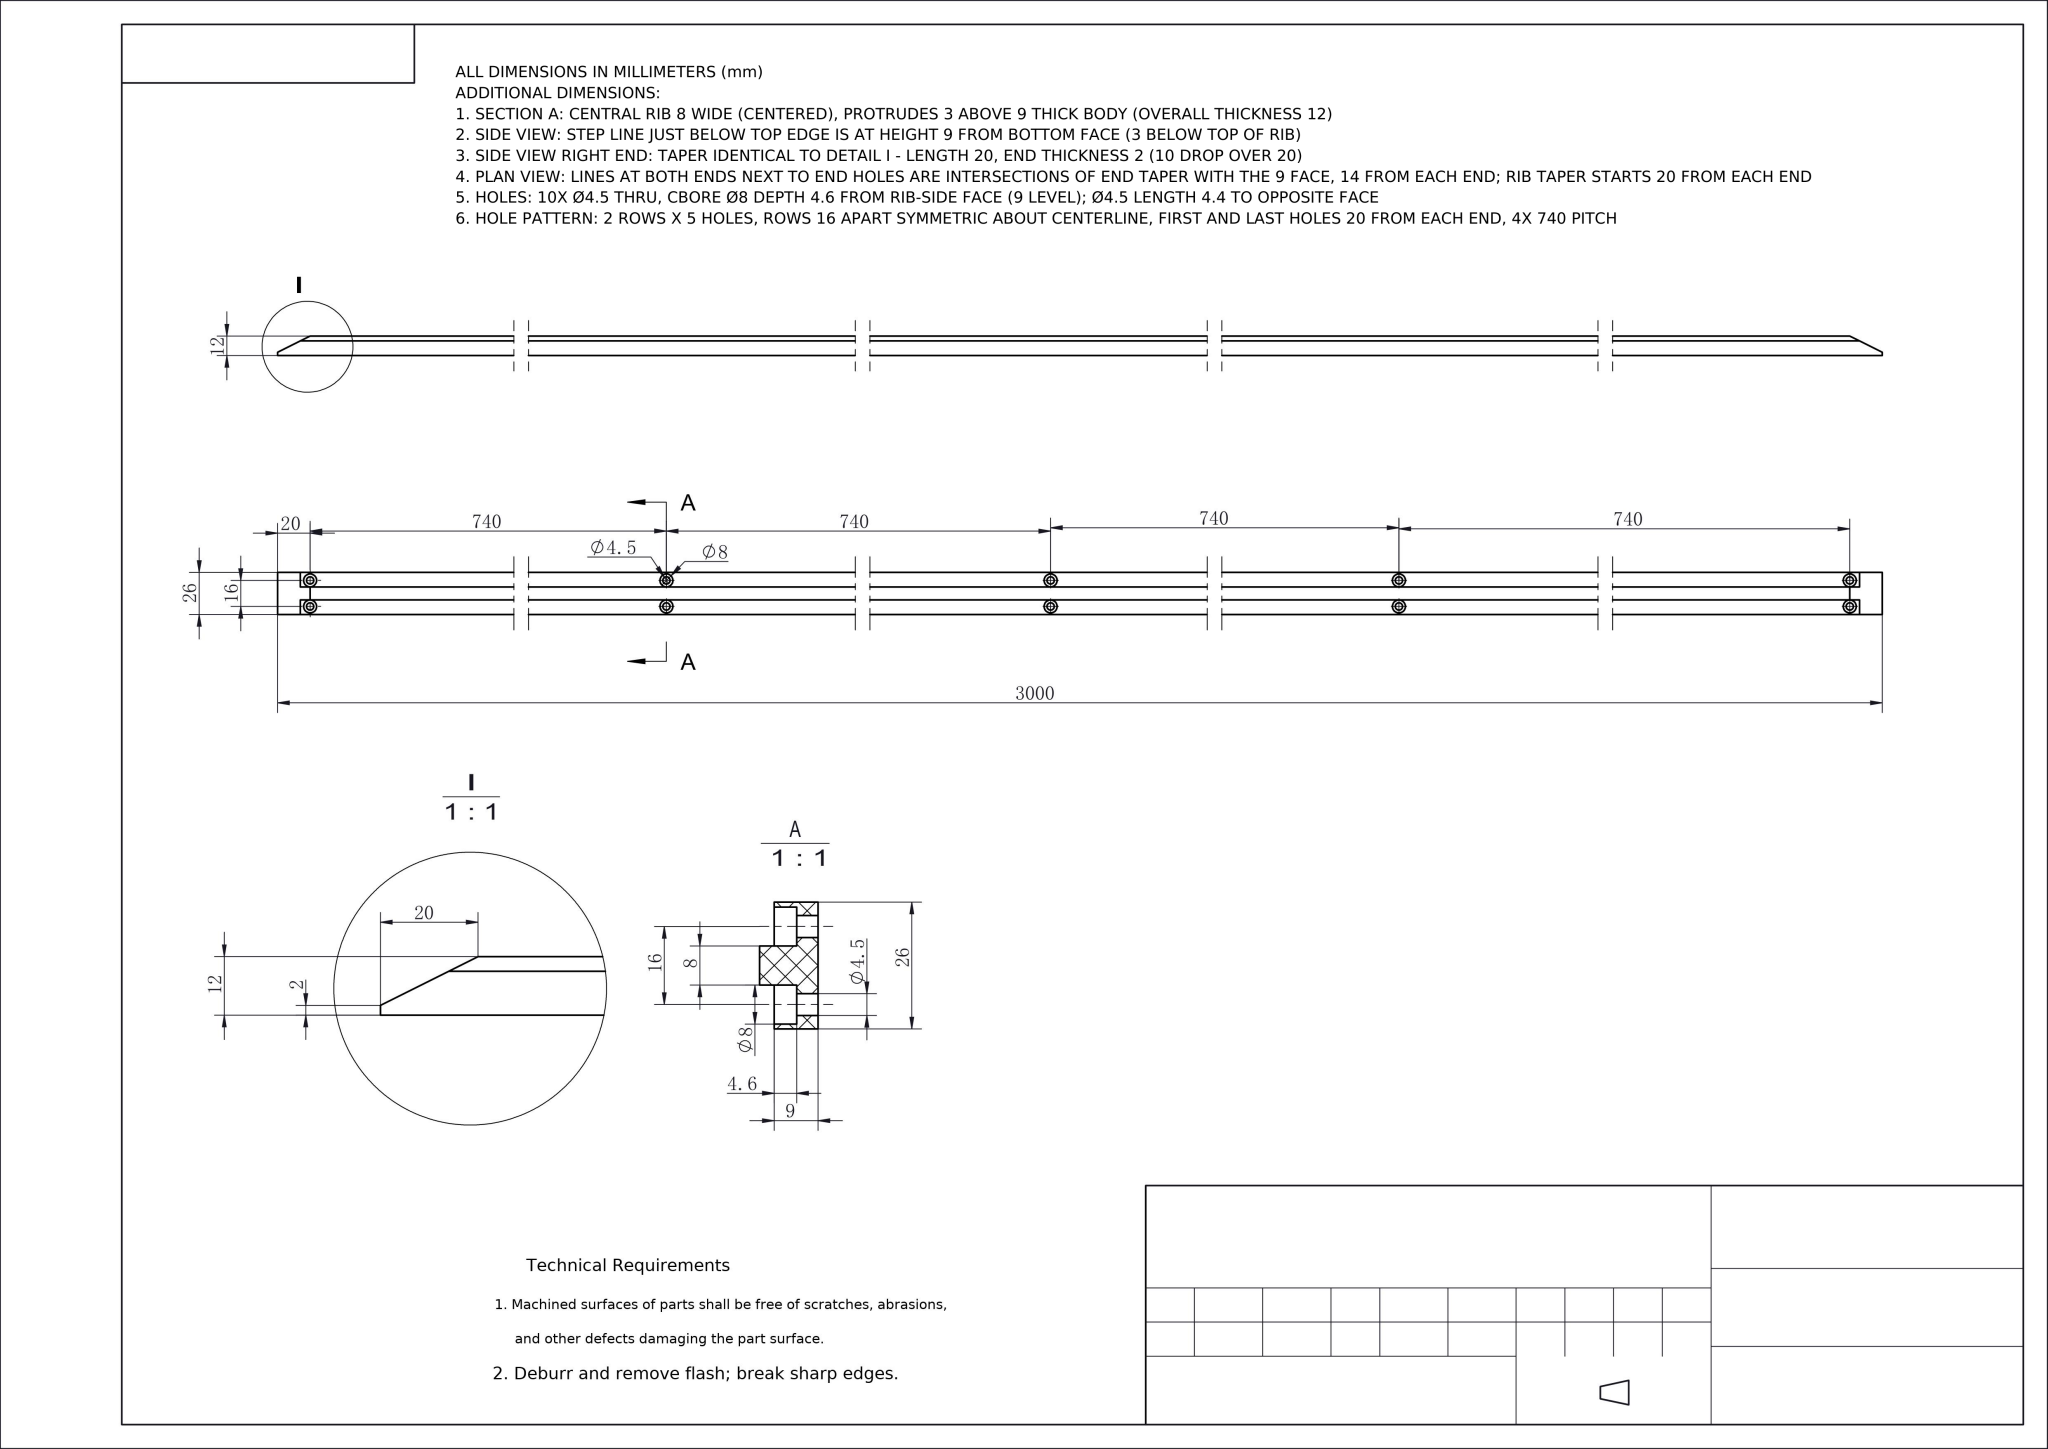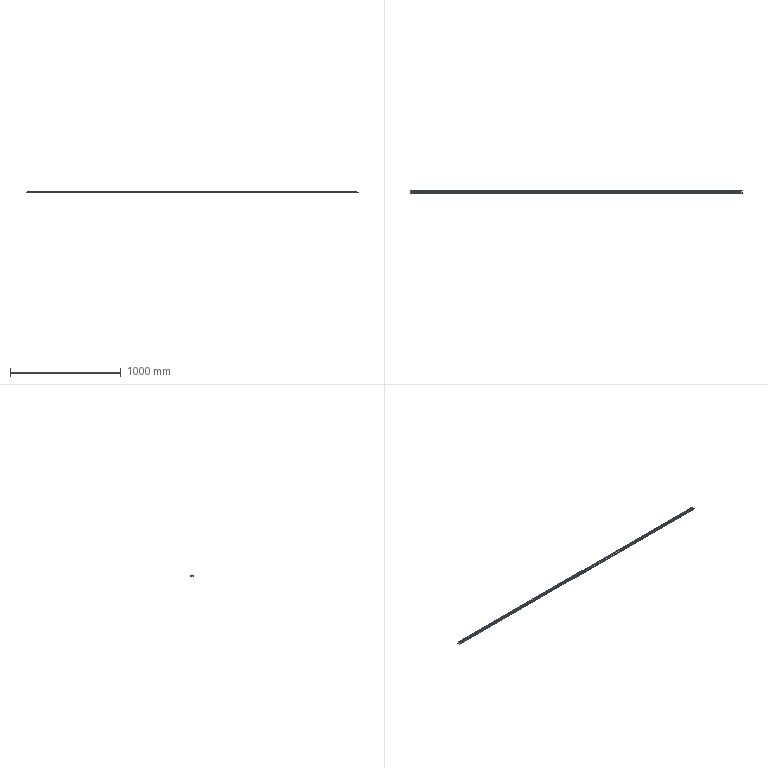Part | NX | mm | 1 solid | 62 faces | box 3000 x 26 x 12 mm | volume 767624 mm3 | cylinder 40 | plane 22 | commonest cylinder face diameters 8 x20 4.5 x20